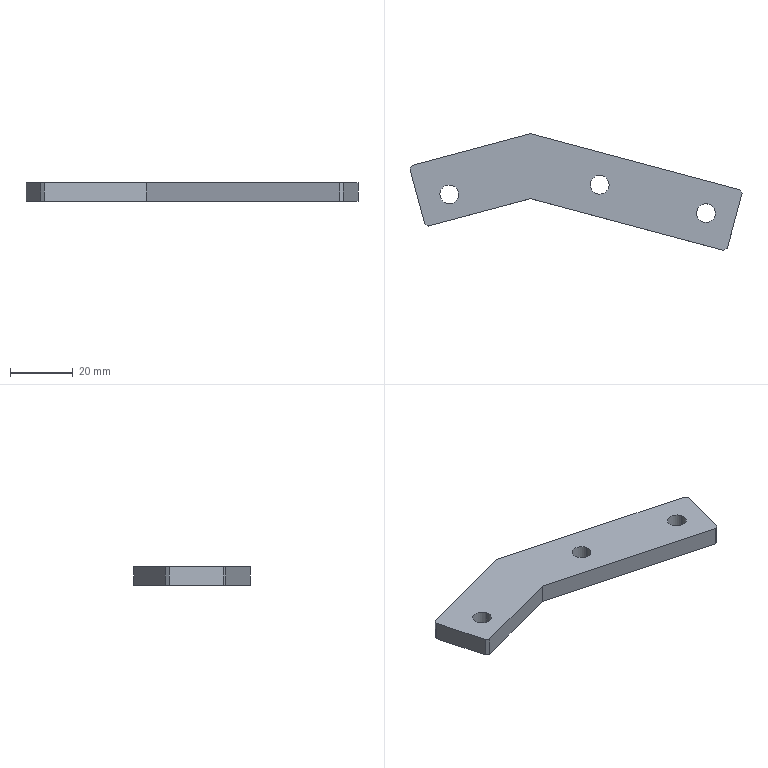Component | SolidWorks | JCT-03-05BentPlate-1 | 1 solid | 18 faces | box 105.73 x 37.18 x 6 mm | volume 12036 mm3 | plane 12 | cylinder 6 | commonest cylinder face diameters 6 x6
build123d program:
from build123d import *

# Parameters (mm, degrees)
EXTRUDE1_DEPTH    = 3
SKETCH2_R         = 3
EXTRUDE2_DEPTH    = 114.57
M6_TAPPED_HOLE1_D = 6
CHAMFER1_SIZE     = 1


with BuildPart() as part:
    # Sketch1 → Extrude1 (new, symmetric)
    with BuildSketch(Plane.XY):
        Polygon((0, 0), (40, 0), (100.622, -35), (90.622, -52.321), (34.641, -20), (0, -20), align=None)
    extrude(amount=EXTRUDE1_DEPTH, both=True)

    # Sketch2 → Extrude2 (cut, through all)
    with BuildSketch(Plane.XY.offset(3)):
        with Locations((10, -12)):
            Circle(SKETCH2_R)
    extrude(amount=-EXTRUDE2_DEPTH, mode=Mode.SUBTRACT)

    # M6 Tapped Hole1 (through all)
    with Locations(Plane.XY.offset(3)):
        with Locations((57.084, -21.41), (87.395, -38.91)):
            Hole(M6_TAPPED_HOLE1_D / 2)

    # Chamfer1
    chamfer1_edges = [part.edges().sort_by_distance(p)[0] for p in [
        (0, 0, 0),
        (100.622, -35, 0),
        (90.622, -52.321, 0),
        (0, -20, 0),
    ]]
    chamfer(chamfer1_edges, length=CHAMFER1_SIZE)


solid = part.part

# Placed as in the assembly
solid = solid.moved(Location((10.501, 12.302, 65), (0, 0, 15)))
STEP:
#1=CARTESIAN_POINT('',(2.688,0.2212,2.441));
#2=VERTEX_POINT('',#1);
#3=CARTESIAN_POINT('',(2.916,0.2824,2.441));
#4=VERTEX_POINT('',#3);
#5=CARTESIAN_POINT('',(2.802,0.2518,2.441));
#6=DIRECTION('',(0.,0.,1.));
#7=DIRECTION('',(0.9659,0.2588,0.));
#8=AXIS2_PLACEMENT_3D('',#5,#6,#7);
#9=CIRCLE('',#8,0.1181);
#10=EDGE_CURVE('',#2,#4,#9,.T.);
#11=ORIENTED_EDGE('',*,*,#10,.F.);
#12=CARTESIAN_POINT('',(2.688,0.2212,2.677));
#13=VERTEX_POINT('',#12);
#14=CARTESIAN_POINT('',(2.688,0.2212,2.677));
#15=DIRECTION('',(0.,0.,1.));
#16=VECTOR('',#15,39.37);
#17=LINE('',#14,#16);
#18=EDGE_CURVE('',#2,#13,#17,.T.);
#19=ORIENTED_EDGE('',*,*,#18,.T.);
#20=CARTESIAN_POINT('',(2.916,0.2824,2.677));
#21=VERTEX_POINT('',#20);
#22=CARTESIAN_POINT('',(2.802,0.2518,2.677));
#23=DIRECTION('',(0.,0.,1.));
#24=DIRECTION('',(0.9659,0.2588,0.));
#25=AXIS2_PLACEMENT_3D('',#22,#23,#24);
#26=CIRCLE('',#25,0.1181);
#27=EDGE_CURVE('',#13,#21,#26,.T.);
#28=ORIENTED_EDGE('',*,*,#27,.T.);
#29=CARTESIAN_POINT('',(2.916,0.2824,2.677));
#30=DIRECTION('',(0.,0.,1.));
#31=VECTOR('',#30,39.37);
#32=LINE('',#29,#31);
#33=EDGE_CURVE('',#4,#21,#32,.T.);
#34=ORIENTED_EDGE('',*,*,#33,.F.);
#35=EDGE_LOOP('',(#11,#19,#28,#34));
#36=FACE_OUTER_BOUND('',#35,.T.);
#37=CARTESIAN_POINT('',(2.802,0.2518,2.677));
#38=DIRECTION('',(0.,0.,1.));
#39=DIRECTION('',(0.9659,0.2588,0.));
#40=AXIS2_PLACEMENT_3D('',#37,#38,#39);
#41=CYLINDRICAL_SURFACE('',#40,0.1181);
#42=ADVANCED_FACE('',(#36),#41,.F.);
#43=CARTESIAN_POINT('',(4.019,-0.1354,2.441));
#44=VERTEX_POINT('',#43);
#45=CARTESIAN_POINT('',(4.247,-0.07427,2.441));
#46=VERTEX_POINT('',#45);
#47=CARTESIAN_POINT('',(4.133,-0.1048,2.441));
#48=DIRECTION('',(0.,0.,1.));
#49=DIRECTION('',(0.9659,0.2588,0.));
#50=AXIS2_PLACEMENT_3D('',#47,#48,#49);
#51=CIRCLE('',#50,0.1181);
#52=EDGE_CURVE('',#44,#46,#51,.T.);
#53=ORIENTED_EDGE('',*,*,#52,.F.);
#54=CARTESIAN_POINT('',(4.019,-0.1354,2.677));
#55=VERTEX_POINT('',#54);
#56=CARTESIAN_POINT('',(4.019,-0.1354,2.677));
#57=DIRECTION('',(0.,0.,1.));
#58=VECTOR('',#57,39.37);
#59=LINE('',#56,#58);
#60=EDGE_CURVE('',#44,#55,#59,.T.);
#61=ORIENTED_EDGE('',*,*,#60,.T.);
#62=CARTESIAN_POINT('',(4.247,-0.07427,2.677));
#63=VERTEX_POINT('',#62);
#64=CARTESIAN_POINT('',(4.133,-0.1048,2.677));
#65=DIRECTION('',(0.,0.,1.));
#66=DIRECTION('',(0.9659,0.2588,0.));
#67=AXIS2_PLACEMENT_3D('',#64,#65,#66);
#68=CIRCLE('',#67,0.1181);
#69=EDGE_CURVE('',#55,#63,#68,.T.);
#70=ORIENTED_EDGE('',*,*,#69,.T.);
#71=CARTESIAN_POINT('',(4.247,-0.07427,2.677));
#72=DIRECTION('',(0.,0.,1.));
#73=VECTOR('',#72,39.37);
#74=LINE('',#71,#73);
#75=EDGE_CURVE('',#46,#63,#74,.T.);
#76=ORIENTED_EDGE('',*,*,#75,.F.);
#77=EDGE_LOOP('',(#53,#61,#70,#76));
#78=FACE_OUTER_BOUND('',#77,.T.);
#79=CARTESIAN_POINT('',(4.133,-0.1048,2.677));
#80=DIRECTION('',(0.,0.,1.));
#81=DIRECTION('',(0.9659,0.2588,0.));
#82=AXIS2_PLACEMENT_3D('',#79,#80,#81);
#83=CYLINDRICAL_SURFACE('',#82,0.1181);
#84=ADVANCED_FACE('',(#78),#83,.F.);
#85=CARTESIAN_POINT('',(0.8019,0.09932,2.441));
#86=VERTEX_POINT('',#85);
#87=CARTESIAN_POINT('',(1.03,0.1605,2.441));
#88=VERTEX_POINT('',#87);
#89=CARTESIAN_POINT('',(0.916,0.1299,2.441));
#90=DIRECTION('',(0.,0.,1.));
#91=DIRECTION('',(0.9659,0.2588,0.));
#92=AXIS2_PLACEMENT_3D('',#89,#90,#91);
#93=CIRCLE('',#92,0.1181);
#94=EDGE_CURVE('',#86,#88,#93,.T.);
#95=ORIENTED_EDGE('',*,*,#94,.F.);
#96=CARTESIAN_POINT('',(0.8019,0.09932,2.677));
#97=VERTEX_POINT('',#96);
#98=CARTESIAN_POINT('',(0.8019,0.09932,2.441));
#99=DIRECTION('',(0.,0.,1.));
#100=VECTOR('',#99,39.37);
#101=LINE('',#98,#100);
#102=EDGE_CURVE('',#86,#97,#101,.T.);
#103=ORIENTED_EDGE('',*,*,#102,.T.);
#104=CARTESIAN_POINT('',(1.03,0.1605,2.677));
#105=VERTEX_POINT('',#104);
#106=CARTESIAN_POINT('',(0.916,0.1299,2.677));
#107=DIRECTION('',(0.,0.,1.));
#108=DIRECTION('',(0.9659,0.2588,0.));
#109=AXIS2_PLACEMENT_3D('',#106,#107,#108);
#110=CIRCLE('',#109,0.1181);
#111=EDGE_CURVE('',#97,#105,#110,.T.);
#112=ORIENTED_EDGE('',*,*,#111,.T.);
#113=CARTESIAN_POINT('',(1.03,0.1605,2.441));
#114=DIRECTION('',(0.,0.,1.));
#115=VECTOR('',#114,39.37);
#116=LINE('',#113,#115);
#117=EDGE_CURVE('',#88,#105,#116,.T.);
#118=ORIENTED_EDGE('',*,*,#117,.F.);
#119=EDGE_LOOP('',(#95,#103,#112,#118));
#120=FACE_OUTER_BOUND('',#119,.T.);
#121=CARTESIAN_POINT('',(0.916,0.1299,2.441));
#122=DIRECTION('',(0.,0.,1.));
#123=DIRECTION('',(0.9659,0.2588,0.));
#124=AXIS2_PLACEMENT_3D('',#121,#122,#123);
#125=CYLINDRICAL_SURFACE('',#124,0.1181);
#126=ADVANCED_FACE('',(#120),#125,.F.);
#127=CARTESIAN_POINT('',(0.4236,0.4463,2.441));
#128=VERTEX_POINT('',#127);
#129=CARTESIAN_POINT('',(0.607,-0.2382,2.441));
#130=VERTEX_POINT('',#129);
#131=CARTESIAN_POINT('',(0.4134,0.4843,2.441));
#132=DIRECTION('',(0.2588,-0.9659,0.));
#133=VECTOR('',#132,39.37);
#134=LINE('',#131,#133);
#135=EDGE_CURVE('',#128,#130,#134,.T.);
#136=ORIENTED_EDGE('',*,*,#135,.T.);
#137=CARTESIAN_POINT('',(0.607,-0.2382,2.677));
#138=VERTEX_POINT('',#137);
#139=CARTESIAN_POINT('',(0.607,-0.2382,2.677));
#140=DIRECTION('',(0.,0.,1.));
#141=VECTOR('',#140,39.37);
#142=LINE('',#139,#141);
#143=EDGE_CURVE('',#130,#138,#142,.T.);
#144=ORIENTED_EDGE('',*,*,#143,.T.);
#145=CARTESIAN_POINT('',(0.4236,0.4463,2.677));
#146=VERTEX_POINT('',#145);
#147=CARTESIAN_POINT('',(0.4134,0.4843,2.677));
#148=DIRECTION('',(0.2588,-0.9659,0.));
#149=VECTOR('',#148,39.37);
#150=LINE('',#147,#149);
#151=EDGE_CURVE('',#146,#138,#150,.T.);
#152=ORIENTED_EDGE('',*,*,#151,.F.);
#153=CARTESIAN_POINT('',(0.4236,0.4463,2.677));
#154=DIRECTION('',(0.,0.,-1.));
#155=VECTOR('',#154,39.37);
#156=LINE('',#153,#155);
#157=EDGE_CURVE('',#146,#128,#156,.T.);
#158=ORIENTED_EDGE('',*,*,#157,.T.);
#159=EDGE_LOOP('',(#136,#144,#152,#158));
#160=FACE_OUTER_BOUND('',#159,.T.);
#161=CARTESIAN_POINT('',(0.4134,0.4843,2.677));
#162=DIRECTION('',(0.9659,0.2588,0.));
#163=DIRECTION('',(-0.2588,0.9659,0.));
#164=AXIS2_PLACEMENT_3D('',#161,#162,#163);
#165=PLANE('',#164);
#166=ADVANCED_FACE('',(#160),#165,.F.);
#167=CARTESIAN_POINT('',(0.6553,-0.266,2.677));
#168=VERTEX_POINT('',#167);
#169=CARTESIAN_POINT('',(1.935,0.07674,2.677));
#170=VERTEX_POINT('',#169);
#171=CARTESIAN_POINT('',(0.6172,-0.2762,2.677));
#172=DIRECTION('',(0.9659,0.2588,0.));
#173=VECTOR('',#172,39.37);
#174=LINE('',#171,#173);
#175=EDGE_CURVE('',#168,#170,#174,.T.);
#176=ORIENTED_EDGE('',*,*,#175,.F.);
#177=CARTESIAN_POINT('',(0.6553,-0.266,2.441));
#178=VERTEX_POINT('',#177);
#179=CARTESIAN_POINT('',(0.6553,-0.266,2.677));
#180=DIRECTION('',(0.,0.,-1.));
#181=VECTOR('',#180,39.37);
#182=LINE('',#179,#181);
#183=EDGE_CURVE('',#168,#178,#182,.T.);
#184=ORIENTED_EDGE('',*,*,#183,.T.);
#185=CARTESIAN_POINT('',(1.935,0.07674,2.441));
#186=VERTEX_POINT('',#185);
#187=CARTESIAN_POINT('',(0.6172,-0.2762,2.441));
#188=DIRECTION('',(0.9659,0.2588,0.));
#189=VECTOR('',#188,39.37);
#190=LINE('',#187,#189);
#191=EDGE_CURVE('',#178,#186,#190,.T.);
#192=ORIENTED_EDGE('',*,*,#191,.T.);
#193=CARTESIAN_POINT('',(1.935,0.07674,2.677));
#194=DIRECTION('',(0.,0.,-1.));
#195=VECTOR('',#194,39.37);
#196=LINE('',#193,#195);
#197=EDGE_CURVE('',#170,#186,#196,.T.);
#198=ORIENTED_EDGE('',*,*,#197,.F.);
#199=EDGE_LOOP('',(#176,#184,#192,#198));
#200=FACE_OUTER_BOUND('',#199,.T.);
#201=CARTESIAN_POINT('',(0.6172,-0.2762,2.677));
#202=DIRECTION('',(-0.2588,0.9659,0.));
#203=DIRECTION('',(0.,0.,1.));
#204=AXIS2_PLACEMENT_3D('',#201,#202,#203);
#205=PLANE('',#204);
#206=ADVANCED_FACE('',(#200),#205,.F.);
#207=CARTESIAN_POINT('',(4.355,-0.5717,2.441));
#208=VERTEX_POINT('',#207);
#209=CARTESIAN_POINT('',(1.935,0.07674,2.441));
#210=DIRECTION('',(0.9659,-0.2588,0.));
#211=VECTOR('',#210,39.37);
#212=LINE('',#209,#211);
#213=EDGE_CURVE('',#186,#208,#212,.T.);
#214=ORIENTED_EDGE('',*,*,#213,.T.);
#215=CARTESIAN_POINT('',(4.355,-0.5717,2.677));
#216=VERTEX_POINT('',#215);
#217=CARTESIAN_POINT('',(4.355,-0.5717,2.677));
#218=DIRECTION('',(0.,0.,1.));
#219=VECTOR('',#218,39.37);
#220=LINE('',#217,#219);
#221=EDGE_CURVE('',#208,#216,#220,.T.);
#222=ORIENTED_EDGE('',*,*,#221,.T.);
#223=CARTESIAN_POINT('',(1.935,0.07674,2.677));
#224=DIRECTION('',(0.9659,-0.2588,0.));
#225=VECTOR('',#224,39.37);
#226=LINE('',#223,#225);
#227=EDGE_CURVE('',#170,#216,#226,.T.);
#228=ORIENTED_EDGE('',*,*,#227,.F.);
#229=ORIENTED_EDGE('',*,*,#197,.T.);
#230=EDGE_LOOP('',(#214,#222,#228,#229));
#231=FACE_OUTER_BOUND('',#230,.T.);
#232=CARTESIAN_POINT('',(1.935,0.07674,2.677));
#233=DIRECTION('',(0.2588,0.9659,0.));
#234=DIRECTION('',(-0.9659,0.2588,0.));
#235=AXIS2_PLACEMENT_3D('',#232,#233,#234);
#236=PLANE('',#235);
#237=ADVANCED_FACE('',(#231),#236,.F.);
#238=CARTESIAN_POINT('',(4.403,-0.5439,2.677));
#239=VERTEX_POINT('',#238);
#240=CARTESIAN_POINT('',(4.586,0.1406,2.677));
#241=VERTEX_POINT('',#240);
#242=CARTESIAN_POINT('',(4.393,-0.5819,2.677));
#243=DIRECTION('',(0.2588,0.9659,0.));
#244=VECTOR('',#243,39.37);
#245=LINE('',#242,#244);
#246=EDGE_CURVE('',#239,#241,#245,.T.);
#247=ORIENTED_EDGE('',*,*,#246,.F.);
#248=CARTESIAN_POINT('',(4.403,-0.5439,2.441));
#249=VERTEX_POINT('',#248);
#250=CARTESIAN_POINT('',(4.403,-0.5439,2.677));
#251=DIRECTION('',(0.,0.,-1.));
#252=VECTOR('',#251,39.37);
#253=LINE('',#250,#252);
#254=EDGE_CURVE('',#239,#249,#253,.T.);
#255=ORIENTED_EDGE('',*,*,#254,.T.);
#256=CARTESIAN_POINT('',(4.586,0.1406,2.441));
#257=VERTEX_POINT('',#256);
#258=CARTESIAN_POINT('',(4.393,-0.5819,2.441));
#259=DIRECTION('',(0.2588,0.9659,0.));
#260=VECTOR('',#259,39.37);
#261=LINE('',#258,#260);
#262=EDGE_CURVE('',#249,#257,#261,.T.);
#263=ORIENTED_EDGE('',*,*,#262,.T.);
#264=CARTESIAN_POINT('',(4.586,0.1406,2.677));
#265=DIRECTION('',(0.,0.,1.));
#266=VECTOR('',#265,39.37);
#267=LINE('',#264,#266);
#268=EDGE_CURVE('',#257,#241,#267,.T.);
#269=ORIENTED_EDGE('',*,*,#268,.T.);
#270=EDGE_LOOP('',(#247,#255,#263,#269));
#271=FACE_OUTER_BOUND('',#270,.T.);
#272=CARTESIAN_POINT('',(4.393,-0.5819,2.677));
#273=DIRECTION('',(-0.9659,0.2588,0.));
#274=DIRECTION('',(-0.2588,-0.9659,0.));
#275=AXIS2_PLACEMENT_3D('',#272,#273,#274);
#276=PLANE('',#275);
#277=ADVANCED_FACE('',(#271),#276,.F.);
#278=CARTESIAN_POINT('',(4.559,0.1888,2.677));
#279=VERTEX_POINT('',#278);
#280=CARTESIAN_POINT('',(1.935,0.8919,2.677));
#281=VERTEX_POINT('',#280);
#282=CARTESIAN_POINT('',(1.935,0.8919,2.677));
#283=DIRECTION('',(-0.9659,0.2588,0.));
#284=VECTOR('',#283,39.37);
#285=LINE('',#282,#284);
#286=EDGE_CURVE('',#279,#281,#285,.T.);
#287=ORIENTED_EDGE('',*,*,#286,.F.);
#288=CARTESIAN_POINT('',(4.559,0.1888,2.441));
#289=VERTEX_POINT('',#288);
#290=CARTESIAN_POINT('',(4.559,0.1888,2.677));
#291=DIRECTION('',(0.,0.,-1.));
#292=VECTOR('',#291,39.37);
#293=LINE('',#290,#292);
#294=EDGE_CURVE('',#279,#289,#293,.T.);
#295=ORIENTED_EDGE('',*,*,#294,.T.);
#296=CARTESIAN_POINT('',(1.935,0.8919,2.441));
#297=VERTEX_POINT('',#296);
#298=CARTESIAN_POINT('',(1.935,0.8919,2.441));
#299=DIRECTION('',(-0.9659,0.2588,0.));
#300=VECTOR('',#299,39.37);
#301=LINE('',#298,#300);
#302=EDGE_CURVE('',#289,#297,#301,.T.);
#303=ORIENTED_EDGE('',*,*,#302,.T.);
#304=CARTESIAN_POINT('',(1.935,0.8919,2.677));
#305=DIRECTION('',(0.,0.,-1.));
#306=VECTOR('',#305,39.37);
#307=LINE('',#304,#306);
#308=EDGE_CURVE('',#281,#297,#307,.T.);
#309=ORIENTED_EDGE('',*,*,#308,.F.);
#310=EDGE_LOOP('',(#287,#295,#303,#309));
#311=FACE_OUTER_BOUND('',#310,.T.);
#312=CARTESIAN_POINT('',(1.935,0.8919,2.677));
#313=DIRECTION('',(-0.2588,-0.9659,0.));
#314=DIRECTION('',(0.9659,-0.2588,0.));
#315=AXIS2_PLACEMENT_3D('',#312,#313,#314);
#316=PLANE('',#315);
#317=ADVANCED_FACE('',(#311),#316,.F.);
#318=CARTESIAN_POINT('',(0.4515,0.4945,2.441));
#319=VERTEX_POINT('',#318);
#320=CARTESIAN_POINT('',(0.4134,0.4843,2.441));
#321=DIRECTION('',(-0.9659,-0.2588,0.));
#322=VECTOR('',#321,39.37);
#323=LINE('',#320,#322);
#324=EDGE_CURVE('',#297,#319,#323,.T.);
#325=ORIENTED_EDGE('',*,*,#324,.T.);
#326=CARTESIAN_POINT('',(0.4515,0.4945,2.677));
#327=VERTEX_POINT('',#326);
#328=CARTESIAN_POINT('',(0.4515,0.4945,2.677));
#329=DIRECTION('',(0.,0.,1.));
#330=VECTOR('',#329,39.37);
#331=LINE('',#328,#330);
#332=EDGE_CURVE('',#319,#327,#331,.T.);
#333=ORIENTED_EDGE('',*,*,#332,.T.);
#334=CARTESIAN_POINT('',(0.4134,0.4843,2.677));
#335=DIRECTION('',(-0.9659,-0.2588,0.));
#336=VECTOR('',#335,39.37);
#337=LINE('',#334,#336);
#338=EDGE_CURVE('',#281,#327,#337,.T.);
#339=ORIENTED_EDGE('',*,*,#338,.F.);
#340=ORIENTED_EDGE('',*,*,#308,.T.);
#341=EDGE_LOOP('',(#325,#333,#339,#340));
#342=FACE_OUTER_BOUND('',#341,.T.);
#343=CARTESIAN_POINT('',(0.4134,0.4843,2.677));
#344=DIRECTION('',(0.2588,-0.9659,0.));
#345=DIRECTION('',(0.,0.,-1.));
#346=AXIS2_PLACEMENT_3D('',#343,#344,#345);
#347=PLANE('',#346);
#348=ADVANCED_FACE('',(#342),#347,.F.);
#349=CARTESIAN_POINT('',(2.802,0.2518,2.677));
#350=DIRECTION('',(0.,0.,1.));
#351=DIRECTION('',(0.9659,0.2588,0.));
#352=AXIS2_PLACEMENT_3D('',#349,#350,#351);
#353=CIRCLE('',#352,0.1181);
#354=EDGE_CURVE('',#21,#13,#353,.T.);
#355=ORIENTED_EDGE('',*,*,#354,.F.);
#356=ORIENTED_EDGE('',*,*,#27,.F.);
#357=EDGE_LOOP('',(#355,#356));
#358=FACE_BOUND('',#357,.T.);
#359=CARTESIAN_POINT('',(4.133,-0.1048,2.677));
#360=DIRECTION('',(0.,0.,1.));
#361=DIRECTION('',(0.9659,0.2588,0.));
#362=AXIS2_PLACEMENT_3D('',#359,#360,#361);
#363=CIRCLE('',#362,0.1181);
#364=EDGE_CURVE('',#63,#55,#363,.T.);
#365=ORIENTED_EDGE('',*,*,#364,.F.);
#366=ORIENTED_EDGE('',*,*,#69,.F.);
#367=EDGE_LOOP('',(#365,#366));
#368=FACE_BOUND('',#367,.T.);
#369=CARTESIAN_POINT('',(0.916,0.1299,2.677));
#370=DIRECTION('',(0.,0.,1.));
#371=DIRECTION('',(0.9659,0.2588,0.));
#372=AXIS2_PLACEMENT_3D('',#369,#370,#371);
#373=CIRCLE('',#372,0.1181);
#374=EDGE_CURVE('',#105,#97,#373,.T.);
#375=ORIENTED_EDGE('',*,*,#374,.F.);
#376=ORIENTED_EDGE('',*,*,#111,.F.);
#377=EDGE_LOOP('',(#375,#376));
#378=FACE_BOUND('',#377,.T.);
#379=ORIENTED_EDGE('',*,*,#227,.T.);
#380=CARTESIAN_POINT('',(1.68,-2.116,2.677));
#381=DIRECTION('',(0.866,0.5,0.));
#382=VECTOR('',#381,39.37);
#383=LINE('',#380,#382);
#384=EDGE_CURVE('',#216,#239,#383,.T.);
#385=ORIENTED_EDGE('',*,*,#384,.T.);
#386=ORIENTED_EDGE('',*,*,#246,.T.);
#387=CARTESIAN_POINT('',(3.775,1.547,2.677));
#388=DIRECTION('',(-0.5,0.866,0.));
#389=VECTOR('',#388,39.37);
#390=LINE('',#387,#389);
#391=EDGE_CURVE('',#241,#279,#390,.T.);
#392=ORIENTED_EDGE('',*,*,#391,.T.);
#393=ORIENTED_EDGE('',*,*,#286,.T.);
#394=ORIENTED_EDGE('',*,*,#338,.T.);
#395=CARTESIAN_POINT('',(0.1592,-0.01177,2.677));
#396=DIRECTION('',(-0.5,-0.866,0.));
#397=VECTOR('',#396,39.37);
#398=LINE('',#395,#397);
#399=EDGE_CURVE('',#327,#146,#398,.T.);
#400=ORIENTED_EDGE('',*,*,#399,.T.);
#401=ORIENTED_EDGE('',*,*,#151,.T.);
#402=CARTESIAN_POINT('',(0.6311,-0.2521,2.677));
#403=DIRECTION('',(0.866,-0.5,0.));
#404=VECTOR('',#403,39.37);
#405=LINE('',#402,#404);
#406=EDGE_CURVE('',#138,#168,#405,.T.);
#407=ORIENTED_EDGE('',*,*,#406,.T.);
#408=ORIENTED_EDGE('',*,*,#175,.T.);
#409=EDGE_LOOP('',(#379,#385,#386,#392,#393,#394,#400,#401,#407,#408));
#410=FACE_OUTER_BOUND('',#409,.T.);
#411=CARTESIAN_POINT('',(0.6172,-0.2762,2.677));
#412=DIRECTION('',(0.,0.,1.));
#413=DIRECTION('',(0.9659,0.2588,0.));
#414=AXIS2_PLACEMENT_3D('',#411,#412,#413);
#415=PLANE('',#414);
#416=ADVANCED_FACE('',(#358,#368,#378,#410),#415,.T.);
#417=CARTESIAN_POINT('',(2.802,0.2518,2.441));
#418=DIRECTION('',(0.,0.,1.));
#419=DIRECTION('',(0.9659,0.2588,0.));
#420=AXIS2_PLACEMENT_3D('',#417,#418,#419);
#421=CIRCLE('',#420,0.1181);
#422=EDGE_CURVE('',#4,#2,#421,.T.);
#423=ORIENTED_EDGE('',*,*,#422,.T.);
#424=ORIENTED_EDGE('',*,*,#10,.T.);
#425=EDGE_LOOP('',(#423,#424));
#426=FACE_BOUND('',#425,.T.);
#427=CARTESIAN_POINT('',(4.133,-0.1048,2.441));
#428=DIRECTION('',(0.,0.,1.));
#429=DIRECTION('',(0.9659,0.2588,0.));
#430=AXIS2_PLACEMENT_3D('',#427,#428,#429);
#431=CIRCLE('',#430,0.1181);
#432=EDGE_CURVE('',#46,#44,#431,.T.);
#433=ORIENTED_EDGE('',*,*,#432,.T.);
#434=ORIENTED_EDGE('',*,*,#52,.T.);
#435=EDGE_LOOP('',(#433,#434));
#436=FACE_BOUND('',#435,.T.);
#437=CARTESIAN_POINT('',(0.916,0.1299,2.441));
#438=DIRECTION('',(0.,0.,1.));
#439=DIRECTION('',(0.9659,0.2588,0.));
#440=AXIS2_PLACEMENT_3D('',#437,#438,#439);
#441=CIRCLE('',#440,0.1181);
#442=EDGE_CURVE('',#88,#86,#441,.T.);
#443=ORIENTED_EDGE('',*,*,#442,.T.);
#444=ORIENTED_EDGE('',*,*,#94,.T.);
#445=EDGE_LOOP('',(#443,#444));
#446=FACE_BOUND('',#445,.T.);
#447=ORIENTED_EDGE('',*,*,#262,.F.);
#448=CARTESIAN_POINT('',(4.403,-0.5439,2.441));
#449=DIRECTION('',(-0.866,-0.5,0.));
#450=VECTOR('',#449,39.37);
#451=LINE('',#448,#450);
#452=EDGE_CURVE('',#249,#208,#451,.T.);
#453=ORIENTED_EDGE('',*,*,#452,.T.);
#454=ORIENTED_EDGE('',*,*,#213,.F.);
#455=ORIENTED_EDGE('',*,*,#191,.F.);
#456=CARTESIAN_POINT('',(0.6553,-0.266,2.441));
#457=DIRECTION('',(-0.866,0.5,0.));
#458=VECTOR('',#457,39.37);
#459=LINE('',#456,#458);
#460=EDGE_CURVE('',#178,#130,#459,.T.);
#461=ORIENTED_EDGE('',*,*,#460,.T.);
#462=ORIENTED_EDGE('',*,*,#135,.F.);
#463=CARTESIAN_POINT('',(0.4236,0.4463,2.441));
#464=DIRECTION('',(0.5,0.866,0.));
#465=VECTOR('',#464,39.37);
#466=LINE('',#463,#465);
#467=EDGE_CURVE('',#128,#319,#466,.T.);
#468=ORIENTED_EDGE('',*,*,#467,.T.);
#469=ORIENTED_EDGE('',*,*,#324,.F.);
#470=ORIENTED_EDGE('',*,*,#302,.F.);
#471=CARTESIAN_POINT('',(4.559,0.1888,2.441));
#472=DIRECTION('',(0.5,-0.866,0.));
#473=VECTOR('',#472,39.37);
#474=LINE('',#471,#473);
#475=EDGE_CURVE('',#289,#257,#474,.T.);
#476=ORIENTED_EDGE('',*,*,#475,.T.);
#477=EDGE_LOOP('',(#447,#453,#454,#455,#461,#462,#468,#469,#470,#476));
#478=FACE_OUTER_BOUND('',#477,.T.);
#479=CARTESIAN_POINT('',(0.6172,-0.2762,2.441));
#480=DIRECTION('',(0.,0.,1.));
#481=DIRECTION('',(0.9659,0.2588,0.));
#482=AXIS2_PLACEMENT_3D('',#479,#480,#481);
#483=PLANE('',#482);
#484=ADVANCED_FACE('',(#426,#436,#446,#478),#483,.F.);
#485=ORIENTED_EDGE('',*,*,#102,.F.);
#486=ORIENTED_EDGE('',*,*,#442,.F.);
#487=ORIENTED_EDGE('',*,*,#117,.T.);
#488=ORIENTED_EDGE('',*,*,#374,.T.);
#489=EDGE_LOOP('',(#485,#486,#487,#488));
#490=FACE_OUTER_BOUND('',#489,.T.);
#491=CARTESIAN_POINT('',(0.916,0.1299,2.441));
#492=DIRECTION('',(0.,0.,1.));
#493=DIRECTION('',(0.9659,0.2588,0.));
#494=AXIS2_PLACEMENT_3D('',#491,#492,#493);
#495=CYLINDRICAL_SURFACE('',#494,0.1181);
#496=ADVANCED_FACE('',(#490),#495,.F.);
#497=ORIENTED_EDGE('',*,*,#60,.F.);
#498=ORIENTED_EDGE('',*,*,#432,.F.);
#499=ORIENTED_EDGE('',*,*,#75,.T.);
#500=ORIENTED_EDGE('',*,*,#364,.T.);
#501=EDGE_LOOP('',(#497,#498,#499,#500));
#502=FACE_OUTER_BOUND('',#501,.T.);
#503=CARTESIAN_POINT('',(4.133,-0.1048,2.677));
#504=DIRECTION('',(0.,0.,1.));
#505=DIRECTION('',(0.9659,0.2588,0.));
#506=AXIS2_PLACEMENT_3D('',#503,#504,#505);
#507=CYLINDRICAL_SURFACE('',#506,0.1181);
#508=ADVANCED_FACE('',(#502),#507,.F.);
#509=ORIENTED_EDGE('',*,*,#18,.F.);
#510=ORIENTED_EDGE('',*,*,#422,.F.);
#511=ORIENTED_EDGE('',*,*,#33,.T.);
#512=ORIENTED_EDGE('',*,*,#354,.T.);
#513=EDGE_LOOP('',(#509,#510,#511,#512));
#514=FACE_OUTER_BOUND('',#513,.T.);
#515=CARTESIAN_POINT('',(2.802,0.2518,2.677));
#516=DIRECTION('',(0.,0.,1.));
#517=DIRECTION('',(0.9659,0.2588,0.));
#518=AXIS2_PLACEMENT_3D('',#515,#516,#517);
#519=CYLINDRICAL_SURFACE('',#518,0.1181);
#520=ADVANCED_FACE('',(#514),#519,.F.);
#521=ORIENTED_EDGE('',*,*,#384,.F.);
#522=ORIENTED_EDGE('',*,*,#221,.F.);
#523=ORIENTED_EDGE('',*,*,#452,.F.);
#524=ORIENTED_EDGE('',*,*,#254,.F.);
#525=EDGE_LOOP('',(#521,#522,#523,#524));
#526=FACE_OUTER_BOUND('',#525,.T.);
#527=CARTESIAN_POINT('',(4.403,-0.5439,2.677));
#528=DIRECTION('',(-0.5,0.866,0.));
#529=DIRECTION('',(-0.866,-0.5,0.));
#530=AXIS2_PLACEMENT_3D('',#527,#528,#529);
#531=PLANE('',#530);
#532=ADVANCED_FACE('',(#526),#531,.F.);
#533=ORIENTED_EDGE('',*,*,#391,.F.);
#534=ORIENTED_EDGE('',*,*,#268,.F.);
#535=ORIENTED_EDGE('',*,*,#475,.F.);
#536=ORIENTED_EDGE('',*,*,#294,.F.);
#537=EDGE_LOOP('',(#533,#534,#535,#536));
#538=FACE_OUTER_BOUND('',#537,.T.);
#539=CARTESIAN_POINT('',(4.559,0.1888,2.677));
#540=DIRECTION('',(-0.866,-0.5,0.));
#541=DIRECTION('',(0.5,-0.866,0.));
#542=AXIS2_PLACEMENT_3D('',#539,#540,#541);
#543=PLANE('',#542);
#544=ADVANCED_FACE('',(#538),#543,.F.);
#545=ORIENTED_EDGE('',*,*,#406,.F.);
#546=ORIENTED_EDGE('',*,*,#143,.F.);
#547=ORIENTED_EDGE('',*,*,#460,.F.);
#548=ORIENTED_EDGE('',*,*,#183,.F.);
#549=EDGE_LOOP('',(#545,#546,#547,#548));
#550=FACE_OUTER_BOUND('',#549,.T.);
#551=CARTESIAN_POINT('',(0.6553,-0.266,2.677));
#552=DIRECTION('',(0.5,0.866,0.));
#553=DIRECTION('',(-0.866,0.5,0.));
#554=AXIS2_PLACEMENT_3D('',#551,#552,#553);
#555=PLANE('',#554);
#556=ADVANCED_FACE('',(#550),#555,.F.);
#557=ORIENTED_EDGE('',*,*,#399,.F.);
#558=ORIENTED_EDGE('',*,*,#332,.F.);
#559=ORIENTED_EDGE('',*,*,#467,.F.);
#560=ORIENTED_EDGE('',*,*,#157,.F.);
#561=EDGE_LOOP('',(#557,#558,#559,#560));
#562=FACE_OUTER_BOUND('',#561,.T.);
#563=CARTESIAN_POINT('',(0.4236,0.4463,2.677));
#564=DIRECTION('',(0.866,-0.5,0.));
#565=DIRECTION('',(0.5,0.866,0.));
#566=AXIS2_PLACEMENT_3D('',#563,#564,#565);
#567=PLANE('',#566);
#568=ADVANCED_FACE('',(#562),#567,.F.);
#569=CLOSED_SHELL('',(#42,#84,#126,#166,#206,#237,#277,#317,#348,#416,#484,#496,#508,#520,#532,#544,#556,#568));
#570=MANIFOLD_SOLID_BREP('',#569);
#571=CARTESIAN_POINT('',(0.,0.,0.));
#572=DIRECTION('',(0.,0.,1.));
#573=DIRECTION('',(1.,0.,0.));
#574=AXIS2_PLACEMENT_3D('',#571,#572,#573);
#575=(LENGTH_UNIT()NAMED_UNIT(*)SI_UNIT($,.METRE.));
#576=LENGTH_MEASURE_WITH_UNIT(LENGTH_MEASURE(0.0254),#575);
#577=DIMENSIONAL_EXPONENTS(1.,0.,0.,0.,0.,0.,0.);
#578=(CONVERSION_BASED_UNIT('',#576)LENGTH_UNIT()NAMED_UNIT(#577));
#579=UNCERTAINTY_MEASURE_WITH_UNIT(LENGTH_MEASURE(0.00001),#578,'','');
#580=(NAMED_UNIT(*)PLANE_ANGLE_UNIT()SI_UNIT($,.RADIAN.));
#581=(NAMED_UNIT(*)SI_UNIT($,.STERADIAN.)SOLID_ANGLE_UNIT());
#582=(GEOMETRIC_REPRESENTATION_CONTEXT(3)GLOBAL_UNCERTAINTY_ASSIGNED_CONTEXT((#579))GLOBAL_UNIT_ASSIGNED_CONTEXT((#578,#580,#581))REPRESENTATION_CONTEXT('',''));
#583=ADVANCED_BREP_SHAPE_REPRESENTATION('',(#570,#574),#582);
#584=COLOUR_RGB('',0.7922,0.8196,0.9333);
#585=FILL_AREA_STYLE_COLOUR('',#584);
#586=FILL_AREA_STYLE('',(#585));
#587=SURFACE_STYLE_FILL_AREA(#586);
#588=SURFACE_SIDE_STYLE('',(#587));
#589=SURFACE_STYLE_USAGE(.BOTH.,#588);
#590=PRESENTATION_STYLE_ASSIGNMENT((#589));
#591=STYLED_ITEM('',(#590),#570);
#592=(LENGTH_UNIT()NAMED_UNIT(*)SI_UNIT($,.METRE.));
#593=LENGTH_MEASURE_WITH_UNIT(LENGTH_MEASURE(0.0254),#592);
#594=DIMENSIONAL_EXPONENTS(1.,0.,0.,0.,0.,0.,0.);
#595=(CONVERSION_BASED_UNIT('',#593)LENGTH_UNIT()NAMED_UNIT(#594));
#596=UNCERTAINTY_MEASURE_WITH_UNIT(LENGTH_MEASURE(0.00001),#595,'','');
#597=(NAMED_UNIT(*)PLANE_ANGLE_UNIT()SI_UNIT($,.RADIAN.));
#598=(NAMED_UNIT(*)SI_UNIT($,.STERADIAN.)SOLID_ANGLE_UNIT());
#599=(GEOMETRIC_REPRESENTATION_CONTEXT(3)GLOBAL_UNCERTAINTY_ASSIGNED_CONTEXT((#596))GLOBAL_UNIT_ASSIGNED_CONTEXT((#595,#597,#598))REPRESENTATION_CONTEXT('',''));
#600=MECHANICAL_DESIGN_GEOMETRIC_PRESENTATION_REPRESENTATION('',(#591),#599);
#601=PRESENTATION_LAYER_ASSIGNMENT('','',(#591));